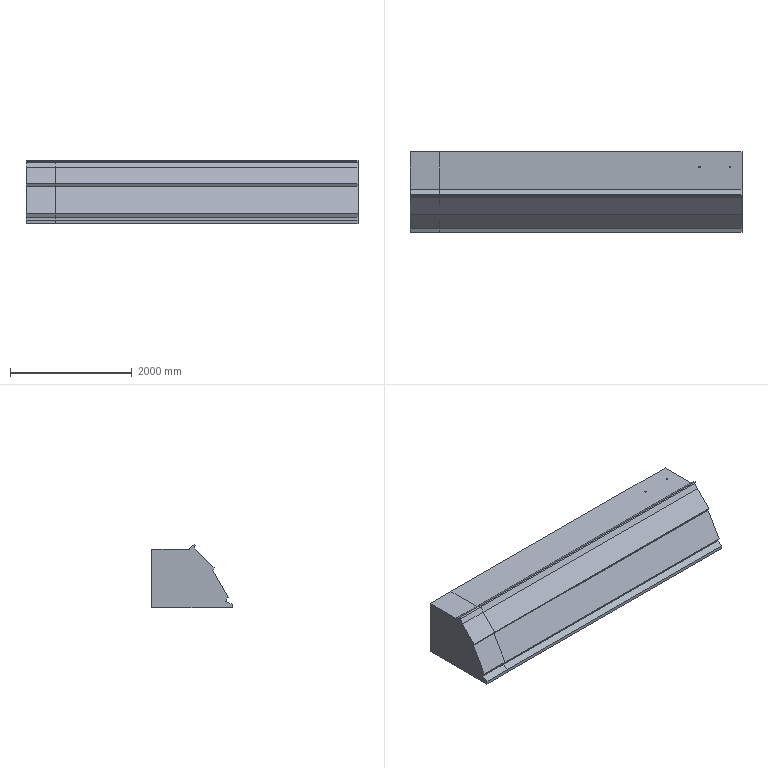Component | NX | SIM15_MASCHINENBETT | 2 solids | 38 faces | volume 5589485629 mm3 | plane 36 | cylinder 2 | commonest cylinder face diameters 25 x2